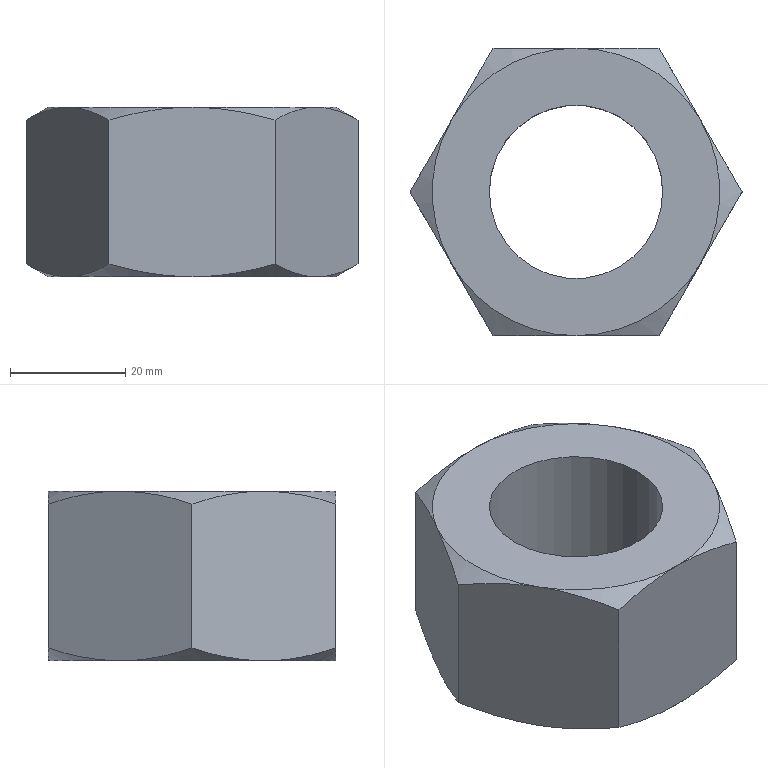Component | NX | GB-T41-2000_M33X3_5 | 1 solid | 21 faces | volume 42521 mm3 | cone 12 | plane 8 | cylinder 1 | commonest cylinder face diameters 30.158 x1